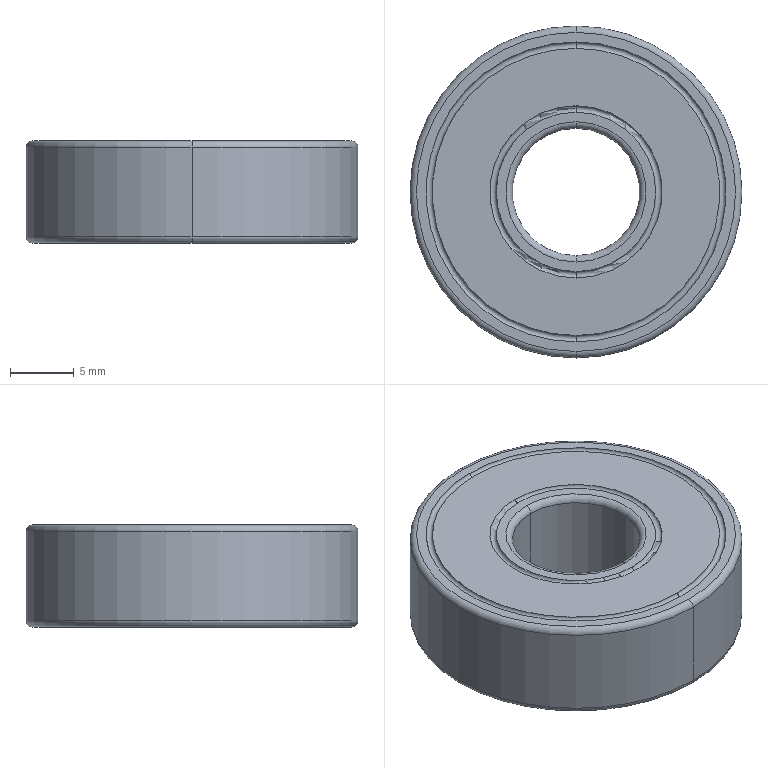Component | SolidWorks | --MA18S200416000Bearing-3 | 1 solid | 26 faces | box 26 x 26 x 8 mm | volume 3585 mm3 | torus 16 | plane 6 | cylinder 4 | commonest cylinder face diameters 10 x2 26 x2
build123d program:
from build123d import *

# Parameters (mm, degrees)
FILLET1_R = 0.5


with BuildPart() as part:
    # Sketch2 → Revolve1 (revolve)
    with BuildSketch(Plane.XY, mode=Mode.PRIVATE) as revolve1_sk:
        with BuildLine():
            Line((6.25, 8), (5, 8))
            Line((5, 8), (5, 0))
            Line((5, 0), (6.25, 0))
            ThreePointArc((6.25, 0), (6.5, 0.25), (6.75, 0))
            Line((6.75, 0), (11.25, 0))
            ThreePointArc((11.25, 0), (11.5, 0.25), (11.75, 0))
            Line((11.75, 0), (13, 0))
            Line((13, 0), (13, 8))
            Line((13, 8), (11.75, 8))
            ThreePointArc((11.75, 8), (11.5, 7.75), (11.25, 8))
            Line((11.25, 8), (6.75, 8))
            ThreePointArc((6.75, 8), (6.5, 7.75), (6.25, 8))
        make_face()
    revolve(revolve1_sk.sketch.rotate(Axis((0, 0, 0), (0, 1, 0)), 90), axis=Axis((0, 0, 0), (0, 1, 0)))

    # Fillet1
    fillet1_edges = [part.edges().sort_by_distance(p)[0] for p in [
        (0, 0, 5),
        (0, 8, 5),
        (0, 8, 13),
        (0, 0, 13),
    ]]
    fillet(fillet1_edges, radius=FILLET1_R)


solid = part.part

# Placed as in the assembly
solid = solid.moved(Location((132.044, 38.699, 21), (90, 0, 0)))
STEP:
#1=CARTESIAN_POINT('',(5.199,2.035,1.122));
#2=VERTEX_POINT('',#1);
#3=CARTESIAN_POINT('',(5.199,1.012,1.122));
#4=VERTEX_POINT('',#3);
#5=CARTESIAN_POINT('',(5.199,1.524,1.122));
#6=DIRECTION('',(0.,-0.,-1.));
#7=DIRECTION('',(0.,-1.,0.));
#8=AXIS2_PLACEMENT_3D('',#5,#6,#7);
#9=CIRCLE('',#8,0.5118);
#10=EDGE_CURVE('',#2,#4,#9,.T.);
#11=ORIENTED_EDGE('',*,*,#10,.F.);
#12=CARTESIAN_POINT('',(5.199,2.016,1.142));
#13=VERTEX_POINT('',#12);
#14=CARTESIAN_POINT('',(5.199,2.016,1.122));
#15=DIRECTION('',(1.,-0.,0.));
#16=DIRECTION('',(0.,1.,0.));
#17=AXIS2_PLACEMENT_3D('',#14,#15,#16);
#18=CIRCLE('',#17,0.01969);
#19=EDGE_CURVE('',#2,#13,#18,.T.);
#20=ORIENTED_EDGE('',*,*,#19,.T.);
#21=CARTESIAN_POINT('',(5.199,1.031,1.142));
#22=VERTEX_POINT('',#21);
#23=CARTESIAN_POINT('',(5.199,1.524,1.142));
#24=DIRECTION('',(0.,0.,1.));
#25=DIRECTION('',(0.,-1.,0.));
#26=AXIS2_PLACEMENT_3D('',#23,#24,#25);
#27=CIRCLE('',#26,0.4921);
#28=EDGE_CURVE('',#22,#13,#27,.T.);
#29=ORIENTED_EDGE('',*,*,#28,.F.);
#30=CARTESIAN_POINT('',(5.199,1.031,1.122));
#31=DIRECTION('',(-1.,0.,0.));
#32=DIRECTION('',(0.,0.,1.));
#33=AXIS2_PLACEMENT_3D('',#30,#31,#32);
#34=CIRCLE('',#33,0.01969);
#35=EDGE_CURVE('',#4,#22,#34,.T.);
#36=ORIENTED_EDGE('',*,*,#35,.F.);
#37=EDGE_LOOP('',(#11,#20,#29,#36));
#38=FACE_OUTER_BOUND('',#37,.T.);
#39=CARTESIAN_POINT('',(5.199,1.524,1.122));
#40=DIRECTION('',(0.,0.,1.));
#41=DIRECTION('',(0.,-1.,0.));
#42=AXIS2_PLACEMENT_3D('',#39,#40,#41);
#43=TOROIDAL_SURFACE('',#42,0.4921,0.01969);
#44=ADVANCED_FACE('',(#38),#43,.T.);
#45=CARTESIAN_POINT('',(5.199,1.012,0.8465));
#46=VERTEX_POINT('',#45);
#47=CARTESIAN_POINT('',(5.199,2.035,0.8465));
#48=VERTEX_POINT('',#47);
#49=CARTESIAN_POINT('',(5.199,1.524,0.8465));
#50=DIRECTION('',(0.,0.,1.));
#51=DIRECTION('',(0.,1.,-0.));
#52=AXIS2_PLACEMENT_3D('',#49,#50,#51);
#53=CIRCLE('',#52,0.5118);
#54=EDGE_CURVE('',#46,#48,#53,.T.);
#55=ORIENTED_EDGE('',*,*,#54,.F.);
#56=CARTESIAN_POINT('',(5.199,1.031,0.8268));
#57=VERTEX_POINT('',#56);
#58=CARTESIAN_POINT('',(5.199,1.031,0.8465));
#59=DIRECTION('',(1.,0.,-0.));
#60=DIRECTION('',(0.,1.,0.));
#61=AXIS2_PLACEMENT_3D('',#58,#59,#60);
#62=CIRCLE('',#61,0.01969);
#63=EDGE_CURVE('',#46,#57,#62,.T.);
#64=ORIENTED_EDGE('',*,*,#63,.T.);
#65=CARTESIAN_POINT('',(5.199,2.016,0.8268));
#66=VERTEX_POINT('',#65);
#67=CARTESIAN_POINT('',(5.199,1.524,0.8268));
#68=DIRECTION('',(0.,-0.,-1.));
#69=DIRECTION('',(0.,1.,-0.));
#70=AXIS2_PLACEMENT_3D('',#67,#68,#69);
#71=CIRCLE('',#70,0.4921);
#72=EDGE_CURVE('',#66,#57,#71,.T.);
#73=ORIENTED_EDGE('',*,*,#72,.F.);
#74=CARTESIAN_POINT('',(5.199,2.016,0.8465));
#75=DIRECTION('',(-1.,0.,0.));
#76=DIRECTION('',(0.,0.,1.));
#77=AXIS2_PLACEMENT_3D('',#74,#75,#76);
#78=CIRCLE('',#77,0.01969);
#79=EDGE_CURVE('',#48,#66,#78,.T.);
#80=ORIENTED_EDGE('',*,*,#79,.F.);
#81=EDGE_LOOP('',(#55,#64,#73,#80));
#82=FACE_OUTER_BOUND('',#81,.T.);
#83=CARTESIAN_POINT('',(5.199,1.524,0.8465));
#84=DIRECTION('',(0.,-0.,-1.));
#85=DIRECTION('',(0.,1.,-0.));
#86=AXIS2_PLACEMENT_3D('',#83,#84,#85);
#87=TOROIDAL_SURFACE('',#86,0.4921,0.01969);
#88=ADVANCED_FACE('',(#82),#87,.T.);
#89=CARTESIAN_POINT('',(5.199,1.74,1.142));
#90=VERTEX_POINT('',#89);
#91=CARTESIAN_POINT('',(5.199,1.307,1.142));
#92=VERTEX_POINT('',#91);
#93=CARTESIAN_POINT('',(5.199,1.524,1.142));
#94=DIRECTION('',(0.,-0.,-1.));
#95=DIRECTION('',(0.,-1.,0.));
#96=AXIS2_PLACEMENT_3D('',#93,#94,#95);
#97=CIRCLE('',#96,0.2165);
#98=EDGE_CURVE('',#90,#92,#97,.T.);
#99=ORIENTED_EDGE('',*,*,#98,.F.);
#100=CARTESIAN_POINT('',(5.199,1.72,1.122));
#101=VERTEX_POINT('',#100);
#102=CARTESIAN_POINT('',(5.199,1.74,1.122));
#103=DIRECTION('',(1.,-0.,0.));
#104=DIRECTION('',(0.,1.,0.));
#105=AXIS2_PLACEMENT_3D('',#102,#103,#104);
#106=CIRCLE('',#105,0.01969);
#107=EDGE_CURVE('',#90,#101,#106,.T.);
#108=ORIENTED_EDGE('',*,*,#107,.T.);
#109=CARTESIAN_POINT('',(5.199,1.327,1.122));
#110=VERTEX_POINT('',#109);
#111=CARTESIAN_POINT('',(5.199,1.524,1.122));
#112=DIRECTION('',(0.,0.,1.));
#113=DIRECTION('',(0.,-1.,0.));
#114=AXIS2_PLACEMENT_3D('',#111,#112,#113);
#115=CIRCLE('',#114,0.1969);
#116=EDGE_CURVE('',#110,#101,#115,.T.);
#117=ORIENTED_EDGE('',*,*,#116,.F.);
#118=CARTESIAN_POINT('',(5.199,1.307,1.122));
#119=DIRECTION('',(-1.,0.,0.));
#120=DIRECTION('',(0.,0.,1.));
#121=AXIS2_PLACEMENT_3D('',#118,#119,#120);
#122=CIRCLE('',#121,0.01969);
#123=EDGE_CURVE('',#92,#110,#122,.T.);
#124=ORIENTED_EDGE('',*,*,#123,.F.);
#125=EDGE_LOOP('',(#99,#108,#117,#124));
#126=FACE_OUTER_BOUND('',#125,.T.);
#127=CARTESIAN_POINT('',(5.199,1.524,1.122));
#128=DIRECTION('',(0.,0.,1.));
#129=DIRECTION('',(0.,-1.,0.));
#130=AXIS2_PLACEMENT_3D('',#127,#128,#129);
#131=TOROIDAL_SURFACE('',#130,0.2165,0.01969);
#132=ADVANCED_FACE('',(#126),#131,.T.);
#133=CARTESIAN_POINT('',(5.199,1.307,0.8268));
#134=VERTEX_POINT('',#133);
#135=CARTESIAN_POINT('',(5.199,1.74,0.8268));
#136=VERTEX_POINT('',#135);
#137=CARTESIAN_POINT('',(5.199,1.524,0.8268));
#138=DIRECTION('',(0.,0.,1.));
#139=DIRECTION('',(0.,1.,-0.));
#140=AXIS2_PLACEMENT_3D('',#137,#138,#139);
#141=CIRCLE('',#140,0.2165);
#142=EDGE_CURVE('',#134,#136,#141,.T.);
#143=ORIENTED_EDGE('',*,*,#142,.F.);
#144=CARTESIAN_POINT('',(5.199,1.327,0.8465));
#145=VERTEX_POINT('',#144);
#146=CARTESIAN_POINT('',(5.199,1.307,0.8465));
#147=DIRECTION('',(1.,0.,-0.));
#148=DIRECTION('',(0.,1.,0.));
#149=AXIS2_PLACEMENT_3D('',#146,#147,#148);
#150=CIRCLE('',#149,0.01969);
#151=EDGE_CURVE('',#134,#145,#150,.T.);
#152=ORIENTED_EDGE('',*,*,#151,.T.);
#153=CARTESIAN_POINT('',(5.199,1.72,0.8465));
#154=VERTEX_POINT('',#153);
#155=CARTESIAN_POINT('',(5.199,1.524,0.8465));
#156=DIRECTION('',(0.,-0.,-1.));
#157=DIRECTION('',(0.,1.,-0.));
#158=AXIS2_PLACEMENT_3D('',#155,#156,#157);
#159=CIRCLE('',#158,0.1969);
#160=EDGE_CURVE('',#154,#145,#159,.T.);
#161=ORIENTED_EDGE('',*,*,#160,.F.);
#162=CARTESIAN_POINT('',(5.199,1.74,0.8465));
#163=DIRECTION('',(-1.,0.,0.));
#164=DIRECTION('',(0.,0.,1.));
#165=AXIS2_PLACEMENT_3D('',#162,#163,#164);
#166=CIRCLE('',#165,0.01969);
#167=EDGE_CURVE('',#136,#154,#166,.T.);
#168=ORIENTED_EDGE('',*,*,#167,.F.);
#169=EDGE_LOOP('',(#143,#152,#161,#168));
#170=FACE_OUTER_BOUND('',#169,.T.);
#171=CARTESIAN_POINT('',(5.199,1.524,0.8465));
#172=DIRECTION('',(0.,-0.,-1.));
#173=DIRECTION('',(0.,1.,-0.));
#174=AXIS2_PLACEMENT_3D('',#171,#172,#173);
#175=TOROIDAL_SURFACE('',#174,0.2165,0.01969);
#176=ADVANCED_FACE('',(#170),#175,.T.);
#177=CARTESIAN_POINT('',(5.199,1.081,0.8268));
#178=VERTEX_POINT('',#177);
#179=CARTESIAN_POINT('',(5.199,1.966,0.8268));
#180=VERTEX_POINT('',#179);
#181=CARTESIAN_POINT('',(5.199,1.524,0.8268));
#182=DIRECTION('',(0.,-0.,-1.));
#183=DIRECTION('',(0.,1.,-0.));
#184=AXIS2_PLACEMENT_3D('',#181,#182,#183);
#185=CIRCLE('',#184,0.4429);
#186=EDGE_CURVE('',#178,#180,#185,.T.);
#187=ORIENTED_EDGE('',*,*,#186,.F.);
#188=CARTESIAN_POINT('',(5.199,1.061,0.8268));
#189=VERTEX_POINT('',#188);
#190=CARTESIAN_POINT('',(5.199,1.071,0.8268));
#191=DIRECTION('',(1.,0.,-0.));
#192=DIRECTION('',(0.,1.,0.));
#193=AXIS2_PLACEMENT_3D('',#190,#191,#192);
#194=CIRCLE('',#193,0.009843);
#195=EDGE_CURVE('',#178,#189,#194,.T.);
#196=ORIENTED_EDGE('',*,*,#195,.T.);
#197=CARTESIAN_POINT('',(5.199,1.986,0.8268));
#198=VERTEX_POINT('',#197);
#199=CARTESIAN_POINT('',(5.199,1.524,0.8268));
#200=DIRECTION('',(0.,-0.,-1.));
#201=DIRECTION('',(0.,1.,-0.));
#202=AXIS2_PLACEMENT_3D('',#199,#200,#201);
#203=CIRCLE('',#202,0.4626);
#204=EDGE_CURVE('',#189,#198,#203,.T.);
#205=ORIENTED_EDGE('',*,*,#204,.T.);
#206=CARTESIAN_POINT('',(5.199,1.976,0.8268));
#207=DIRECTION('',(-1.,0.,0.));
#208=DIRECTION('',(0.,0.,1.));
#209=AXIS2_PLACEMENT_3D('',#206,#207,#208);
#210=CIRCLE('',#209,0.009843);
#211=EDGE_CURVE('',#180,#198,#210,.T.);
#212=ORIENTED_EDGE('',*,*,#211,.F.);
#213=EDGE_LOOP('',(#187,#196,#205,#212));
#214=FACE_OUTER_BOUND('',#213,.T.);
#215=CARTESIAN_POINT('',(5.199,1.524,0.8268));
#216=DIRECTION('',(0.,-0.,-1.));
#217=DIRECTION('',(0.,1.,-0.));
#218=AXIS2_PLACEMENT_3D('',#215,#216,#217);
#219=TOROIDAL_SURFACE('',#218,0.4528,0.009843);
#220=ADVANCED_FACE('',(#214),#219,.F.);
#221=CARTESIAN_POINT('',(5.199,1.278,0.8268));
#222=VERTEX_POINT('',#221);
#223=CARTESIAN_POINT('',(5.199,1.77,0.8268));
#224=VERTEX_POINT('',#223);
#225=CARTESIAN_POINT('',(5.199,1.524,0.8268));
#226=DIRECTION('',(0.,-0.,-1.));
#227=DIRECTION('',(0.,1.,-0.));
#228=AXIS2_PLACEMENT_3D('',#225,#226,#227);
#229=CIRCLE('',#228,0.2461);
#230=EDGE_CURVE('',#222,#224,#229,.T.);
#231=ORIENTED_EDGE('',*,*,#230,.F.);
#232=CARTESIAN_POINT('',(5.199,1.258,0.8268));
#233=VERTEX_POINT('',#232);
#234=CARTESIAN_POINT('',(5.199,1.268,0.8268));
#235=DIRECTION('',(1.,0.,-0.));
#236=DIRECTION('',(0.,1.,0.));
#237=AXIS2_PLACEMENT_3D('',#234,#235,#236);
#238=CIRCLE('',#237,0.009843);
#239=EDGE_CURVE('',#222,#233,#238,.T.);
#240=ORIENTED_EDGE('',*,*,#239,.T.);
#241=CARTESIAN_POINT('',(5.199,1.789,0.8268));
#242=VERTEX_POINT('',#241);
#243=CARTESIAN_POINT('',(5.199,1.524,0.8268));
#244=DIRECTION('',(0.,-0.,-1.));
#245=DIRECTION('',(0.,1.,-0.));
#246=AXIS2_PLACEMENT_3D('',#243,#244,#245);
#247=CIRCLE('',#246,0.2657);
#248=EDGE_CURVE('',#233,#242,#247,.T.);
#249=ORIENTED_EDGE('',*,*,#248,.T.);
#250=CARTESIAN_POINT('',(5.199,1.779,0.8268));
#251=DIRECTION('',(-1.,0.,0.));
#252=DIRECTION('',(0.,0.,1.));
#253=AXIS2_PLACEMENT_3D('',#250,#251,#252);
#254=CIRCLE('',#253,0.009843);
#255=EDGE_CURVE('',#224,#242,#254,.T.);
#256=ORIENTED_EDGE('',*,*,#255,.F.);
#257=EDGE_LOOP('',(#231,#240,#249,#256));
#258=FACE_OUTER_BOUND('',#257,.T.);
#259=CARTESIAN_POINT('',(5.199,1.524,0.8268));
#260=DIRECTION('',(0.,-0.,-1.));
#261=DIRECTION('',(0.,1.,-0.));
#262=AXIS2_PLACEMENT_3D('',#259,#260,#261);
#263=TOROIDAL_SURFACE('',#262,0.2559,0.009843);
#264=ADVANCED_FACE('',(#258),#263,.F.);
#265=CARTESIAN_POINT('',(5.199,1.524,1.122));
#266=DIRECTION('',(0.,0.,1.));
#267=DIRECTION('',(0.,-1.,0.));
#268=AXIS2_PLACEMENT_3D('',#265,#266,#267);
#269=CIRCLE('',#268,0.1969);
#270=EDGE_CURVE('',#101,#110,#269,.T.);
#271=ORIENTED_EDGE('',*,*,#270,.T.);
#272=CARTESIAN_POINT('',(5.199,1.327,0.8268));
#273=DIRECTION('',(0.,-0.,-1.));
#274=VECTOR('',#273,39.37);
#275=LINE('',#272,#274);
#276=EDGE_CURVE('',#110,#145,#275,.T.);
#277=ORIENTED_EDGE('',*,*,#276,.T.);
#278=CARTESIAN_POINT('',(5.199,1.524,0.8465));
#279=DIRECTION('',(0.,-0.,-1.));
#280=DIRECTION('',(0.,1.,-0.));
#281=AXIS2_PLACEMENT_3D('',#278,#279,#280);
#282=CIRCLE('',#281,0.1969);
#283=EDGE_CURVE('',#145,#154,#282,.T.);
#284=ORIENTED_EDGE('',*,*,#283,.T.);
#285=CARTESIAN_POINT('',(5.199,1.72,0.8268));
#286=DIRECTION('',(0.,-0.,-1.));
#287=VECTOR('',#286,39.37);
#288=LINE('',#285,#287);
#289=EDGE_CURVE('',#101,#154,#288,.T.);
#290=ORIENTED_EDGE('',*,*,#289,.F.);
#291=EDGE_LOOP('',(#271,#277,#284,#290));
#292=FACE_OUTER_BOUND('',#291,.T.);
#293=CARTESIAN_POINT('',(5.199,1.524,0.8268));
#294=DIRECTION('',(0.,-0.,-1.));
#295=DIRECTION('',(0.,1.,-0.));
#296=AXIS2_PLACEMENT_3D('',#293,#294,#295);
#297=CYLINDRICAL_SURFACE('',#296,0.1969);
#298=ADVANCED_FACE('',(#292),#297,.F.);
#299=CARTESIAN_POINT('',(5.199,1.258,1.142));
#300=VERTEX_POINT('',#299);
#301=CARTESIAN_POINT('',(5.199,1.789,1.142));
#302=VERTEX_POINT('',#301);
#303=CARTESIAN_POINT('',(5.199,1.524,1.142));
#304=DIRECTION('',(0.,-0.,-1.));
#305=DIRECTION('',(0.,1.,-0.));
#306=AXIS2_PLACEMENT_3D('',#303,#304,#305);
#307=CIRCLE('',#306,0.2657);
#308=EDGE_CURVE('',#300,#302,#307,.T.);
#309=ORIENTED_EDGE('',*,*,#308,.F.);
#310=CARTESIAN_POINT('',(5.199,1.278,1.142));
#311=VERTEX_POINT('',#310);
#312=CARTESIAN_POINT('',(5.199,1.268,1.142));
#313=DIRECTION('',(1.,0.,-0.));
#314=DIRECTION('',(0.,1.,0.));
#315=AXIS2_PLACEMENT_3D('',#312,#313,#314);
#316=CIRCLE('',#315,0.009843);
#317=EDGE_CURVE('',#300,#311,#316,.T.);
#318=ORIENTED_EDGE('',*,*,#317,.T.);
#319=CARTESIAN_POINT('',(5.199,1.77,1.142));
#320=VERTEX_POINT('',#319);
#321=CARTESIAN_POINT('',(5.199,1.524,1.142));
#322=DIRECTION('',(0.,-0.,-1.));
#323=DIRECTION('',(0.,1.,-0.));
#324=AXIS2_PLACEMENT_3D('',#321,#322,#323);
#325=CIRCLE('',#324,0.2461);
#326=EDGE_CURVE('',#311,#320,#325,.T.);
#327=ORIENTED_EDGE('',*,*,#326,.T.);
#328=CARTESIAN_POINT('',(5.199,1.779,1.142));
#329=DIRECTION('',(-1.,0.,0.));
#330=DIRECTION('',(0.,0.,1.));
#331=AXIS2_PLACEMENT_3D('',#328,#329,#330);
#332=CIRCLE('',#331,0.009843);
#333=EDGE_CURVE('',#302,#320,#332,.T.);
#334=ORIENTED_EDGE('',*,*,#333,.F.);
#335=EDGE_LOOP('',(#309,#318,#327,#334));
#336=FACE_OUTER_BOUND('',#335,.T.);
#337=CARTESIAN_POINT('',(5.199,1.524,1.142));
#338=DIRECTION('',(0.,-0.,-1.));
#339=DIRECTION('',(0.,1.,-0.));
#340=AXIS2_PLACEMENT_3D('',#337,#338,#339);
#341=TOROIDAL_SURFACE('',#340,0.2559,0.009843);
#342=ADVANCED_FACE('',(#336),#341,.F.);
#343=CARTESIAN_POINT('',(5.199,1.061,1.142));
#344=VERTEX_POINT('',#343);
#345=CARTESIAN_POINT('',(5.199,1.986,1.142));
#346=VERTEX_POINT('',#345);
#347=CARTESIAN_POINT('',(5.199,1.524,1.142));
#348=DIRECTION('',(0.,-0.,-1.));
#349=DIRECTION('',(0.,1.,-0.));
#350=AXIS2_PLACEMENT_3D('',#347,#348,#349);
#351=CIRCLE('',#350,0.4626);
#352=EDGE_CURVE('',#344,#346,#351,.T.);
#353=ORIENTED_EDGE('',*,*,#352,.F.);
#354=CARTESIAN_POINT('',(5.199,1.081,1.142));
#355=VERTEX_POINT('',#354);
#356=CARTESIAN_POINT('',(5.199,1.071,1.142));
#357=DIRECTION('',(1.,0.,-0.));
#358=DIRECTION('',(0.,1.,0.));
#359=AXIS2_PLACEMENT_3D('',#356,#357,#358);
#360=CIRCLE('',#359,0.009843);
#361=EDGE_CURVE('',#344,#355,#360,.T.);
#362=ORIENTED_EDGE('',*,*,#361,.T.);
#363=CARTESIAN_POINT('',(5.199,1.966,1.142));
#364=VERTEX_POINT('',#363);
#365=CARTESIAN_POINT('',(5.199,1.524,1.142));
#366=DIRECTION('',(0.,-0.,-1.));
#367=DIRECTION('',(0.,1.,-0.));
#368=AXIS2_PLACEMENT_3D('',#365,#366,#367);
#369=CIRCLE('',#368,0.4429);
#370=EDGE_CURVE('',#355,#364,#369,.T.);
#371=ORIENTED_EDGE('',*,*,#370,.T.);
#372=CARTESIAN_POINT('',(5.199,1.976,1.142));
#373=DIRECTION('',(-1.,0.,0.));
#374=DIRECTION('',(0.,0.,1.));
#375=AXIS2_PLACEMENT_3D('',#372,#373,#374);
#376=CIRCLE('',#375,0.009843);
#377=EDGE_CURVE('',#346,#364,#376,.T.);
#378=ORIENTED_EDGE('',*,*,#377,.F.);
#379=EDGE_LOOP('',(#353,#362,#371,#378));
#380=FACE_OUTER_BOUND('',#379,.T.);
#381=CARTESIAN_POINT('',(5.199,1.524,1.142));
#382=DIRECTION('',(0.,-0.,-1.));
#383=DIRECTION('',(0.,1.,-0.));
#384=AXIS2_PLACEMENT_3D('',#381,#382,#383);
#385=TOROIDAL_SURFACE('',#384,0.4528,0.009843);
#386=ADVANCED_FACE('',(#380),#385,.F.);
#387=ORIENTED_EDGE('',*,*,#10,.T.);
#388=CARTESIAN_POINT('',(5.199,1.012,0.8268));
#389=DIRECTION('',(0.,-0.,-1.));
#390=VECTOR('',#389,39.37);
#391=LINE('',#388,#390);
#392=EDGE_CURVE('',#4,#46,#391,.T.);
#393=ORIENTED_EDGE('',*,*,#392,.T.);
#394=ORIENTED_EDGE('',*,*,#54,.T.);
#395=CARTESIAN_POINT('',(5.199,2.035,0.8268));
#396=DIRECTION('',(0.,-0.,-1.));
#397=VECTOR('',#396,39.37);
#398=LINE('',#395,#397);
#399=EDGE_CURVE('',#2,#48,#398,.T.);
#400=ORIENTED_EDGE('',*,*,#399,.F.);
#401=EDGE_LOOP('',(#387,#393,#394,#400));
#402=FACE_OUTER_BOUND('',#401,.T.);
#403=CARTESIAN_POINT('',(5.199,1.524,0.8268));
#404=DIRECTION('',(0.,-0.,-1.));
#405=DIRECTION('',(0.,1.,-0.));
#406=AXIS2_PLACEMENT_3D('',#403,#404,#405);
#407=CYLINDRICAL_SURFACE('',#406,0.5118);
#408=ADVANCED_FACE('',(#402),#407,.T.);
#409=ORIENTED_EDGE('',*,*,#392,.F.);
#410=CARTESIAN_POINT('',(5.199,1.524,1.122));
#411=DIRECTION('',(0.,-0.,-1.));
#412=DIRECTION('',(0.,-1.,0.));
#413=AXIS2_PLACEMENT_3D('',#410,#411,#412);
#414=CIRCLE('',#413,0.5118);
#415=EDGE_CURVE('',#4,#2,#414,.T.);
#416=ORIENTED_EDGE('',*,*,#415,.T.);
#417=ORIENTED_EDGE('',*,*,#399,.T.);
#418=CARTESIAN_POINT('',(5.199,1.524,0.8465));
#419=DIRECTION('',(0.,0.,1.));
#420=DIRECTION('',(0.,1.,-0.));
#421=AXIS2_PLACEMENT_3D('',#418,#419,#420);
#422=CIRCLE('',#421,0.5118);
#423=EDGE_CURVE('',#48,#46,#422,.T.);
#424=ORIENTED_EDGE('',*,*,#423,.T.);
#425=EDGE_LOOP('',(#409,#416,#417,#424));
#426=FACE_OUTER_BOUND('',#425,.T.);
#427=CARTESIAN_POINT('',(5.199,1.524,0.8268));
#428=DIRECTION('',(0.,-0.,-1.));
#429=DIRECTION('',(0.,1.,-0.));
#430=AXIS2_PLACEMENT_3D('',#427,#428,#429);
#431=CYLINDRICAL_SURFACE('',#430,0.5118);
#432=ADVANCED_FACE('',(#426),#431,.T.);
#433=ORIENTED_EDGE('',*,*,#28,.T.);
#434=CARTESIAN_POINT('',(5.199,1.524,1.142));
#435=DIRECTION('',(0.,0.,1.));
#436=DIRECTION('',(0.,-1.,0.));
#437=AXIS2_PLACEMENT_3D('',#434,#435,#436);
#438=CIRCLE('',#437,0.4921);
#439=EDGE_CURVE('',#13,#22,#438,.T.);
#440=ORIENTED_EDGE('',*,*,#439,.T.);
#441=EDGE_LOOP('',(#433,#440));
#442=FACE_OUTER_BOUND('',#441,.T.);
#443=CARTESIAN_POINT('',(5.199,1.524,1.142));
#444=DIRECTION('',(0.,-0.,-1.));
#445=DIRECTION('',(0.,1.,-0.));
#446=AXIS2_PLACEMENT_3D('',#443,#444,#445);
#447=CIRCLE('',#446,0.4626);
#448=EDGE_CURVE('',#346,#344,#447,.T.);
#449=ORIENTED_EDGE('',*,*,#448,.T.);
#450=ORIENTED_EDGE('',*,*,#352,.T.);
#451=EDGE_LOOP('',(#449,#450));
#452=FACE_BOUND('',#451,.T.);
#453=CARTESIAN_POINT('',(5.71,1.524,1.142));
#454=DIRECTION('',(0.,0.,1.));
#455=DIRECTION('',(0.,-1.,0.));
#456=AXIS2_PLACEMENT_3D('',#453,#454,#455);
#457=PLANE('',#456);
#458=ADVANCED_FACE('',(#442,#452),#457,.T.);
#459=ORIENTED_EDGE('',*,*,#361,.F.);
#460=ORIENTED_EDGE('',*,*,#448,.F.);
#461=ORIENTED_EDGE('',*,*,#377,.T.);
#462=CARTESIAN_POINT('',(5.199,1.524,1.142));
#463=DIRECTION('',(0.,-0.,-1.));
#464=DIRECTION('',(0.,1.,-0.));
#465=AXIS2_PLACEMENT_3D('',#462,#463,#464);
#466=CIRCLE('',#465,0.4429);
#467=EDGE_CURVE('',#364,#355,#466,.T.);
#468=ORIENTED_EDGE('',*,*,#467,.T.);
#469=EDGE_LOOP('',(#459,#460,#461,#468));
#470=FACE_OUTER_BOUND('',#469,.T.);
#471=CARTESIAN_POINT('',(5.199,1.524,1.142));
#472=DIRECTION('',(0.,-0.,-1.));
#473=DIRECTION('',(0.,1.,-0.));
#474=AXIS2_PLACEMENT_3D('',#471,#472,#473);
#475=TOROIDAL_SURFACE('',#474,0.4528,0.009843);
#476=ADVANCED_FACE('',(#470),#475,.F.);
#477=CARTESIAN_POINT('',(5.199,1.524,1.142));
#478=DIRECTION('',(0.,-0.,-1.));
#479=DIRECTION('',(0.,1.,-0.));
#480=AXIS2_PLACEMENT_3D('',#477,#478,#479);
#481=CIRCLE('',#480,0.2657);
#482=EDGE_CURVE('',#302,#300,#481,.T.);
#483=ORIENTED_EDGE('',*,*,#482,.T.);
#484=ORIENTED_EDGE('',*,*,#308,.T.);
#485=EDGE_LOOP('',(#483,#484));
#486=FACE_BOUND('',#485,.T.);
#487=ORIENTED_EDGE('',*,*,#467,.F.);
#488=ORIENTED_EDGE('',*,*,#370,.F.);
#489=EDGE_LOOP('',(#487,#488));
#490=FACE_OUTER_BOUND('',#489,.T.);
#491=CARTESIAN_POINT('',(5.641,1.524,1.142));
#492=DIRECTION('',(0.,0.,1.));
#493=DIRECTION('',(0.,-1.,0.));
#494=AXIS2_PLACEMENT_3D('',#491,#492,#493);
#495=PLANE('',#494);
#496=ADVANCED_FACE('',(#486,#490),#495,.T.);
#497=ORIENTED_EDGE('',*,*,#317,.F.);
#498=ORIENTED_EDGE('',*,*,#482,.F.);
#499=ORIENTED_EDGE('',*,*,#333,.T.);
#500=CARTESIAN_POINT('',(5.199,1.524,1.142));
#501=DIRECTION('',(0.,-0.,-1.));
#502=DIRECTION('',(0.,1.,-0.));
#503=AXIS2_PLACEMENT_3D('',#500,#501,#502);
#504=CIRCLE('',#503,0.2461);
#505=EDGE_CURVE('',#320,#311,#504,.T.);
#506=ORIENTED_EDGE('',*,*,#505,.T.);
#507=EDGE_LOOP('',(#497,#498,#499,#506));
#508=FACE_OUTER_BOUND('',#507,.T.);
#509=CARTESIAN_POINT('',(5.199,1.524,1.142));
#510=DIRECTION('',(0.,-0.,-1.));
#511=DIRECTION('',(0.,1.,-0.));
#512=AXIS2_PLACEMENT_3D('',#509,#510,#511);
#513=TOROIDAL_SURFACE('',#512,0.2559,0.009843);
#514=ADVANCED_FACE('',(#508),#513,.F.);
#515=CARTESIAN_POINT('',(5.199,1.524,1.142));
#516=DIRECTION('',(0.,-0.,-1.));
#517=DIRECTION('',(0.,-1.,0.));
#518=AXIS2_PLACEMENT_3D('',#515,#516,#517);
#519=CIRCLE('',#518,0.2165);
#520=EDGE_CURVE('',#92,#90,#519,.T.);
#521=ORIENTED_EDGE('',*,*,#520,.T.);
#522=ORIENTED_EDGE('',*,*,#98,.T.);
#523=EDGE_LOOP('',(#521,#522));
#524=FACE_BOUND('',#523,.T.);
#525=ORIENTED_EDGE('',*,*,#505,.F.);
#526=ORIENTED_EDGE('',*,*,#326,.F.);
#527=EDGE_LOOP('',(#525,#526));
#528=FACE_OUTER_BOUND('',#527,.T.);
#529=CARTESIAN_POINT('',(5.445,1.524,1.142));
#530=DIRECTION('',(0.,0.,1.));
#531=DIRECTION('',(0.,-1.,0.));
#532=AXIS2_PLACEMENT_3D('',#529,#530,#531);
#533=PLANE('',#532);
#534=ADVANCED_FACE('',(#524,#528),#533,.T.);
#535=ORIENTED_EDGE('',*,*,#276,.F.);
#536=ORIENTED_EDGE('',*,*,#116,.T.);
#537=ORIENTED_EDGE('',*,*,#289,.T.);
#538=ORIENTED_EDGE('',*,*,#160,.T.);
#539=EDGE_LOOP('',(#535,#536,#537,#538));
#540=FACE_OUTER_BOUND('',#539,.T.);
#541=CARTESIAN_POINT('',(5.199,1.524,0.8268));
#542=DIRECTION('',(0.,-0.,-1.));
#543=DIRECTION('',(0.,1.,-0.));
#544=AXIS2_PLACEMENT_3D('',#541,#542,#543);
#545=CYLINDRICAL_SURFACE('',#544,0.1969);
#546=ADVANCED_FACE('',(#540),#545,.F.);
#547=CARTESIAN_POINT('',(5.199,1.524,0.8268));
#548=DIRECTION('',(0.,0.,1.));
#549=DIRECTION('',(0.,1.,-0.));
#550=AXIS2_PLACEMENT_3D('',#547,#548,#549);
#551=CIRCLE('',#550,0.2165);
#552=EDGE_CURVE('',#136,#134,#551,.T.);
#553=ORIENTED_EDGE('',*,*,#552,.T.);
#554=ORIENTED_EDGE('',*,*,#142,.T.);
#555=EDGE_LOOP('',(#553,#554));
#556=FACE_BOUND('',#555,.T.);
#557=CARTESIAN_POINT('',(5.199,1.524,0.8268));
#558=DIRECTION('',(0.,-0.,-1.));
#559=DIRECTION('',(0.,1.,-0.));
#560=AXIS2_PLACEMENT_3D('',#557,#558,#559);
#561=CIRCLE('',#560,0.2461);
#562=EDGE_CURVE('',#224,#222,#561,.T.);
#563=ORIENTED_EDGE('',*,*,#562,.T.);
#564=ORIENTED_EDGE('',*,*,#230,.T.);
#565=EDGE_LOOP('',(#563,#564));
#566=FACE_OUTER_BOUND('',#565,.T.);
#567=CARTESIAN_POINT('',(5.445,1.524,0.8268));
#568=DIRECTION('',(0.,-0.,-1.));
#569=DIRECTION('',(0.,1.,-0.));
#570=AXIS2_PLACEMENT_3D('',#567,#568,#569);
#571=PLANE('',#570);
#572=ADVANCED_FACE('',(#556,#566),#571,.T.);
#573=ORIENTED_EDGE('',*,*,#239,.F.);
#574=ORIENTED_EDGE('',*,*,#562,.F.);
#575=ORIENTED_EDGE('',*,*,#255,.T.);
#576=CARTESIAN_POINT('',(5.199,1.524,0.8268));
#577=DIRECTION('',(0.,-0.,-1.));
#578=DIRECTION('',(0.,1.,-0.));
#579=AXIS2_PLACEMENT_3D('',#576,#577,#578);
#580=CIRCLE('',#579,0.2657);
#581=EDGE_CURVE('',#242,#233,#580,.T.);
#582=ORIENTED_EDGE('',*,*,#581,.T.);
#583=EDGE_LOOP('',(#573,#574,#575,#582));
#584=FACE_OUTER_BOUND('',#583,.T.);
#585=CARTESIAN_POINT('',(5.199,1.524,0.8268));
#586=DIRECTION('',(0.,-0.,-1.));
#587=DIRECTION('',(0.,1.,-0.));
#588=AXIS2_PLACEMENT_3D('',#585,#586,#587);
#589=TOROIDAL_SURFACE('',#588,0.2559,0.009843);
#590=ADVANCED_FACE('',(#584),#589,.F.);
#591=CARTESIAN_POINT('',(5.199,1.524,0.8268));
#592=DIRECTION('',(0.,-0.,-1.));
#593=DIRECTION('',(0.,1.,-0.));
#594=AXIS2_PLACEMENT_3D('',#591,#592,#593);
#595=CIRCLE('',#594,0.4429);
#596=EDGE_CURVE('',#180,#178,#595,.T.);
#597=ORIENTED_EDGE('',*,*,#596,.T.);
#598=ORIENTED_EDGE('',*,*,#186,.T.);
#599=EDGE_LOOP('',(#597,#598));
#600=FACE_OUTER_BOUND('',#599,.T.);
#601=ORIENTED_EDGE('',*,*,#581,.F.);
#602=ORIENTED_EDGE('',*,*,#248,.F.);
#603=EDGE_LOOP('',(#601,#602));
#604=FACE_BOUND('',#603,.T.);
#605=CARTESIAN_POINT('',(5.641,1.524,0.8268));
#606=DIRECTION('',(0.,-0.,-1.));
#607=DIRECTION('',(0.,1.,-0.));
#608=AXIS2_PLACEMENT_3D('',#605,#606,#607);
#609=PLANE('',#608);
#610=ADVANCED_FACE('',(#600,#604),#609,.T.);
#611=ORIENTED_EDGE('',*,*,#195,.F.);
#612=ORIENTED_EDGE('',*,*,#596,.F.);
#613=ORIENTED_EDGE('',*,*,#211,.T.);
#614=CARTESIAN_POINT('',(5.199,1.524,0.8268));
#615=DIRECTION('',(0.,-0.,-1.));
#616=DIRECTION('',(0.,1.,-0.));
#617=AXIS2_PLACEMENT_3D('',#614,#615,#616);
#618=CIRCLE('',#617,0.4626);
#619=EDGE_CURVE('',#198,#189,#618,.T.);
#620=ORIENTED_EDGE('',*,*,#619,.T.);
#621=EDGE_LOOP('',(#611,#612,#613,#620));
#622=FACE_OUTER_BOUND('',#621,.T.);
#623=CARTESIAN_POINT('',(5.199,1.524,0.8268));
#624=DIRECTION('',(0.,-0.,-1.));
#625=DIRECTION('',(0.,1.,-0.));
#626=AXIS2_PLACEMENT_3D('',#623,#624,#625);
#627=TOROIDAL_SURFACE('',#626,0.4528,0.009843);
#628=ADVANCED_FACE('',(#622),#627,.F.);
#629=ORIENTED_EDGE('',*,*,#72,.T.);
#630=CARTESIAN_POINT('',(5.199,1.524,0.8268));
#631=DIRECTION('',(0.,-0.,-1.));
#632=DIRECTION('',(0.,1.,-0.));
#633=AXIS2_PLACEMENT_3D('',#630,#631,#632);
#634=CIRCLE('',#633,0.4921);
#635=EDGE_CURVE('',#57,#66,#634,.T.);
#636=ORIENTED_EDGE('',*,*,#635,.T.);
#637=EDGE_LOOP('',(#629,#636));
#638=FACE_OUTER_BOUND('',#637,.T.);
#639=ORIENTED_EDGE('',*,*,#619,.F.);
#640=ORIENTED_EDGE('',*,*,#204,.F.);
#641=EDGE_LOOP('',(#639,#640));
#642=FACE_BOUND('',#641,.T.);
#643=CARTESIAN_POINT('',(5.71,1.524,0.8268));
#644=DIRECTION('',(0.,-0.,-1.));
#645=DIRECTION('',(0.,1.,-0.));
#646=AXIS2_PLACEMENT_3D('',#643,#644,#645);
#647=PLANE('',#646);
#648=ADVANCED_FACE('',(#638,#642),#647,.T.);
#649=ORIENTED_EDGE('',*,*,#151,.F.);
#650=ORIENTED_EDGE('',*,*,#552,.F.);
#651=ORIENTED_EDGE('',*,*,#167,.T.);
#652=ORIENTED_EDGE('',*,*,#283,.F.);
#653=EDGE_LOOP('',(#649,#650,#651,#652));
#654=FACE_OUTER_BOUND('',#653,.T.);
#655=CARTESIAN_POINT('',(5.199,1.524,0.8465));
#656=DIRECTION('',(0.,-0.,-1.));
#657=DIRECTION('',(0.,1.,-0.));
#658=AXIS2_PLACEMENT_3D('',#655,#656,#657);
#659=TOROIDAL_SURFACE('',#658,0.2165,0.01969);
#660=ADVANCED_FACE('',(#654),#659,.T.);
#661=ORIENTED_EDGE('',*,*,#107,.F.);
#662=ORIENTED_EDGE('',*,*,#520,.F.);
#663=ORIENTED_EDGE('',*,*,#123,.T.);
#664=ORIENTED_EDGE('',*,*,#270,.F.);
#665=EDGE_LOOP('',(#661,#662,#663,#664));
#666=FACE_OUTER_BOUND('',#665,.T.);
#667=CARTESIAN_POINT('',(5.199,1.524,1.122));
#668=DIRECTION('',(0.,0.,1.));
#669=DIRECTION('',(0.,-1.,0.));
#670=AXIS2_PLACEMENT_3D('',#667,#668,#669);
#671=TOROIDAL_SURFACE('',#670,0.2165,0.01969);
#672=ADVANCED_FACE('',(#666),#671,.T.);
#673=ORIENTED_EDGE('',*,*,#63,.F.);
#674=ORIENTED_EDGE('',*,*,#423,.F.);
#675=ORIENTED_EDGE('',*,*,#79,.T.);
#676=ORIENTED_EDGE('',*,*,#635,.F.);
#677=EDGE_LOOP('',(#673,#674,#675,#676));
#678=FACE_OUTER_BOUND('',#677,.T.);
#679=CARTESIAN_POINT('',(5.199,1.524,0.8465));
#680=DIRECTION('',(0.,-0.,-1.));
#681=DIRECTION('',(0.,1.,-0.));
#682=AXIS2_PLACEMENT_3D('',#679,#680,#681);
#683=TOROIDAL_SURFACE('',#682,0.4921,0.01969);
#684=ADVANCED_FACE('',(#678),#683,.T.);
#685=ORIENTED_EDGE('',*,*,#19,.F.);
#686=ORIENTED_EDGE('',*,*,#415,.F.);
#687=ORIENTED_EDGE('',*,*,#35,.T.);
#688=ORIENTED_EDGE('',*,*,#439,.F.);
#689=EDGE_LOOP('',(#685,#686,#687,#688));
#690=FACE_OUTER_BOUND('',#689,.T.);
#691=CARTESIAN_POINT('',(5.199,1.524,1.122));
#692=DIRECTION('',(0.,0.,1.));
#693=DIRECTION('',(0.,-1.,0.));
#694=AXIS2_PLACEMENT_3D('',#691,#692,#693);
#695=TOROIDAL_SURFACE('',#694,0.4921,0.01969);
#696=ADVANCED_FACE('',(#690),#695,.T.);
#697=CLOSED_SHELL('',(#44,#88,#132,#176,#220,#264,#298,#342,#386,#408,#432,#458,#476,#496,#514,#534,#546,#572,#590,#610,#628,#648,#660,#672,#684,#696));
#698=MANIFOLD_SOLID_BREP('',#697);
#699=CARTESIAN_POINT('',(0.,0.,0.));
#700=DIRECTION('',(0.,0.,1.));
#701=DIRECTION('',(1.,0.,0.));
#702=AXIS2_PLACEMENT_3D('',#699,#700,#701);
#703=(LENGTH_UNIT()NAMED_UNIT(*)SI_UNIT($,.METRE.));
#704=LENGTH_MEASURE_WITH_UNIT(LENGTH_MEASURE(0.0254),#703);
#705=DIMENSIONAL_EXPONENTS(1.,0.,0.,0.,0.,0.,0.);
#706=(CONVERSION_BASED_UNIT('',#704)LENGTH_UNIT()NAMED_UNIT(#705));
#707=UNCERTAINTY_MEASURE_WITH_UNIT(LENGTH_MEASURE(0.00001),#706,'','');
#708=(NAMED_UNIT(*)PLANE_ANGLE_UNIT()SI_UNIT($,.RADIAN.));
#709=(NAMED_UNIT(*)SI_UNIT($,.STERADIAN.)SOLID_ANGLE_UNIT());
#710=(GEOMETRIC_REPRESENTATION_CONTEXT(3)GLOBAL_UNCERTAINTY_ASSIGNED_CONTEXT((#707))GLOBAL_UNIT_ASSIGNED_CONTEXT((#706,#708,#709))REPRESENTATION_CONTEXT('',''));
#711=ADVANCED_BREP_SHAPE_REPRESENTATION('',(#698,#702),#710);
#712=COLOUR_RGB('',0.7922,0.8196,0.9333);
#713=FILL_AREA_STYLE_COLOUR('',#712);
#714=FILL_AREA_STYLE('',(#713));
#715=SURFACE_STYLE_FILL_AREA(#714);
#716=SURFACE_SIDE_STYLE('',(#715));
#717=SURFACE_STYLE_USAGE(.BOTH.,#716);
#718=PRESENTATION_STYLE_ASSIGNMENT((#717));
#719=STYLED_ITEM('',(#718),#698);
#720=(LENGTH_UNIT()NAMED_UNIT(*)SI_UNIT($,.METRE.));
#721=LENGTH_MEASURE_WITH_UNIT(LENGTH_MEASURE(0.0254),#720);
#722=DIMENSIONAL_EXPONENTS(1.,0.,0.,0.,0.,0.,0.);
#723=(CONVERSION_BASED_UNIT('',#721)LENGTH_UNIT()NAMED_UNIT(#722));
#724=UNCERTAINTY_MEASURE_WITH_UNIT(LENGTH_MEASURE(0.00001),#723,'','');
#725=(NAMED_UNIT(*)PLANE_ANGLE_UNIT()SI_UNIT($,.RADIAN.));
#726=(NAMED_UNIT(*)SI_UNIT($,.STERADIAN.)SOLID_ANGLE_UNIT());
#727=(GEOMETRIC_REPRESENTATION_CONTEXT(3)GLOBAL_UNCERTAINTY_ASSIGNED_CONTEXT((#724))GLOBAL_UNIT_ASSIGNED_CONTEXT((#723,#725,#726))REPRESENTATION_CONTEXT('',''));
#728=MECHANICAL_DESIGN_GEOMETRIC_PRESENTATION_REPRESENTATION('',(#719),#727);
#729=PRESENTATION_LAYER_ASSIGNMENT('','',(#719));